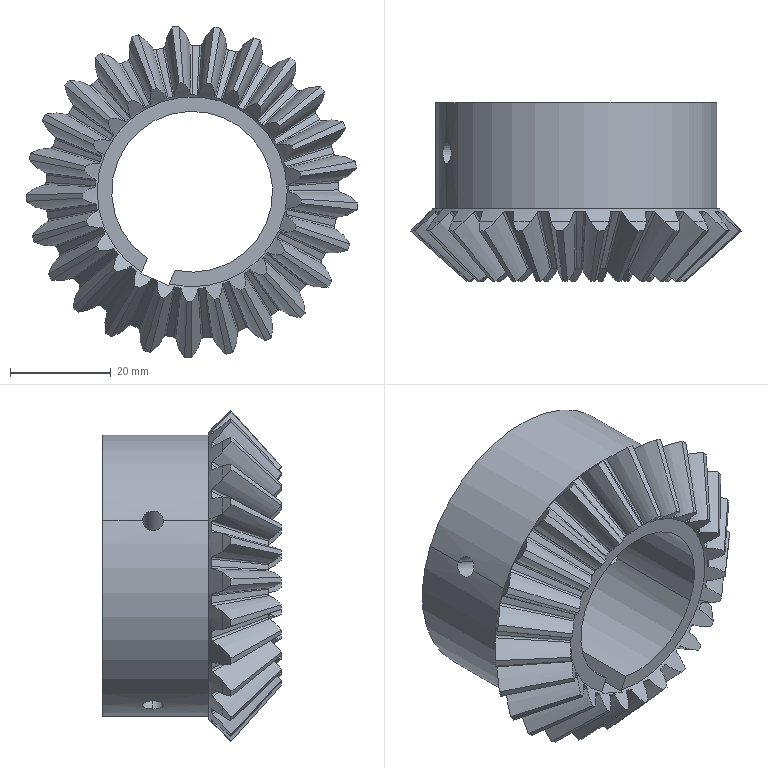Component | SolidWorks | -TractorBevelGear01-1 | 1 solid | 196 faces | volume 52146 mm3 | spline 125 | cone 54 | cylinder 11 | plane 6 | commonest cylinder face diameters 4.2 x6 32 x3 56 x2